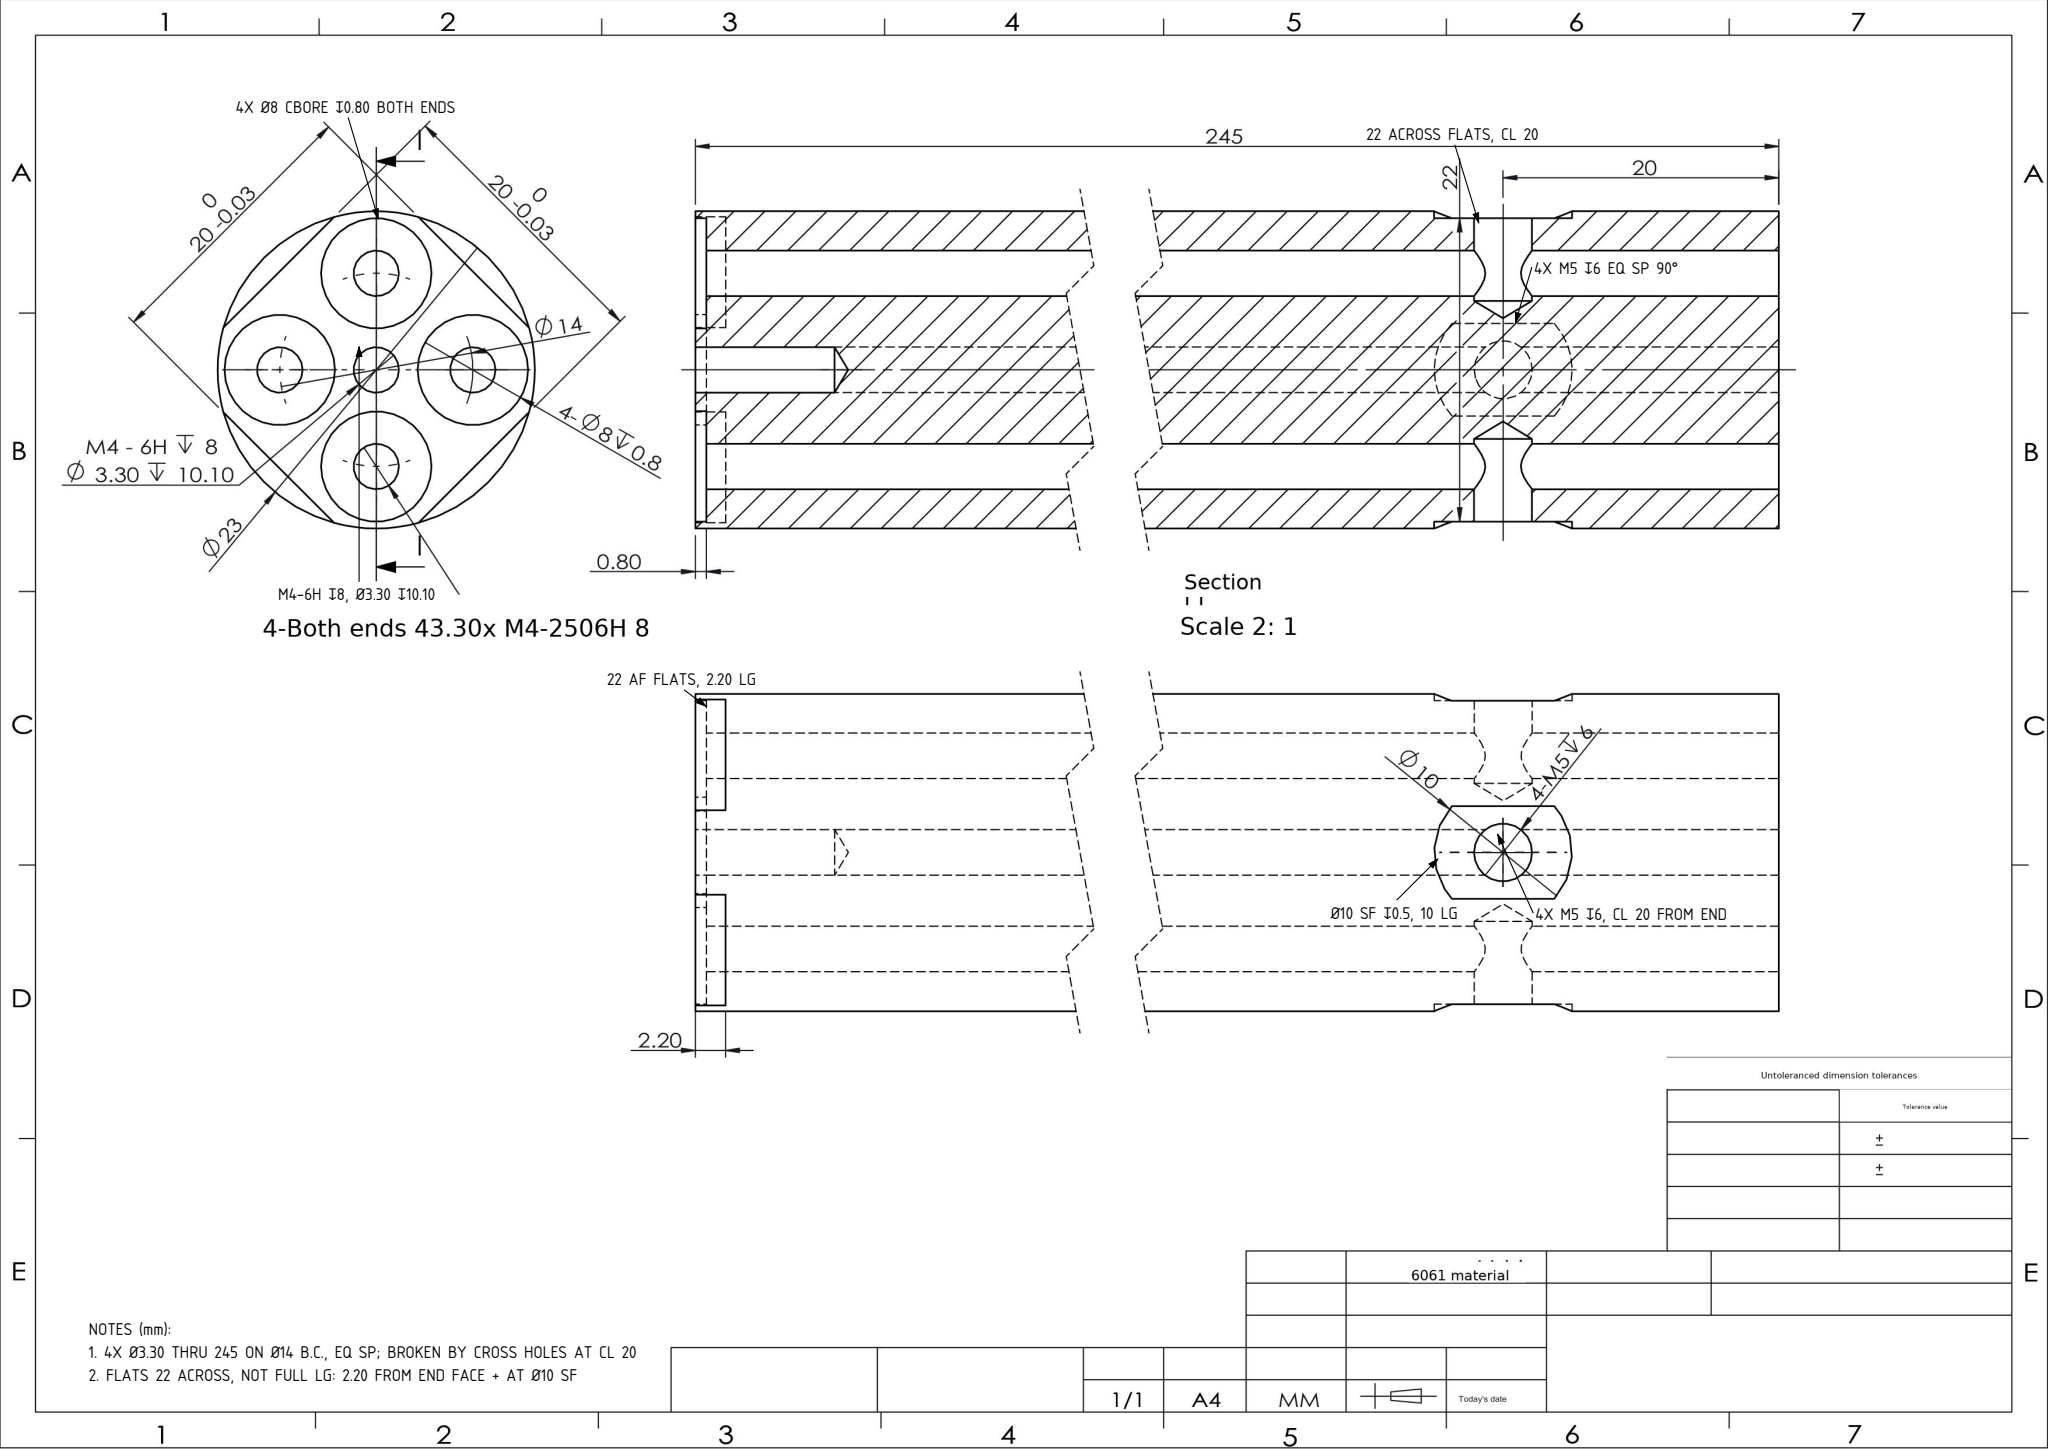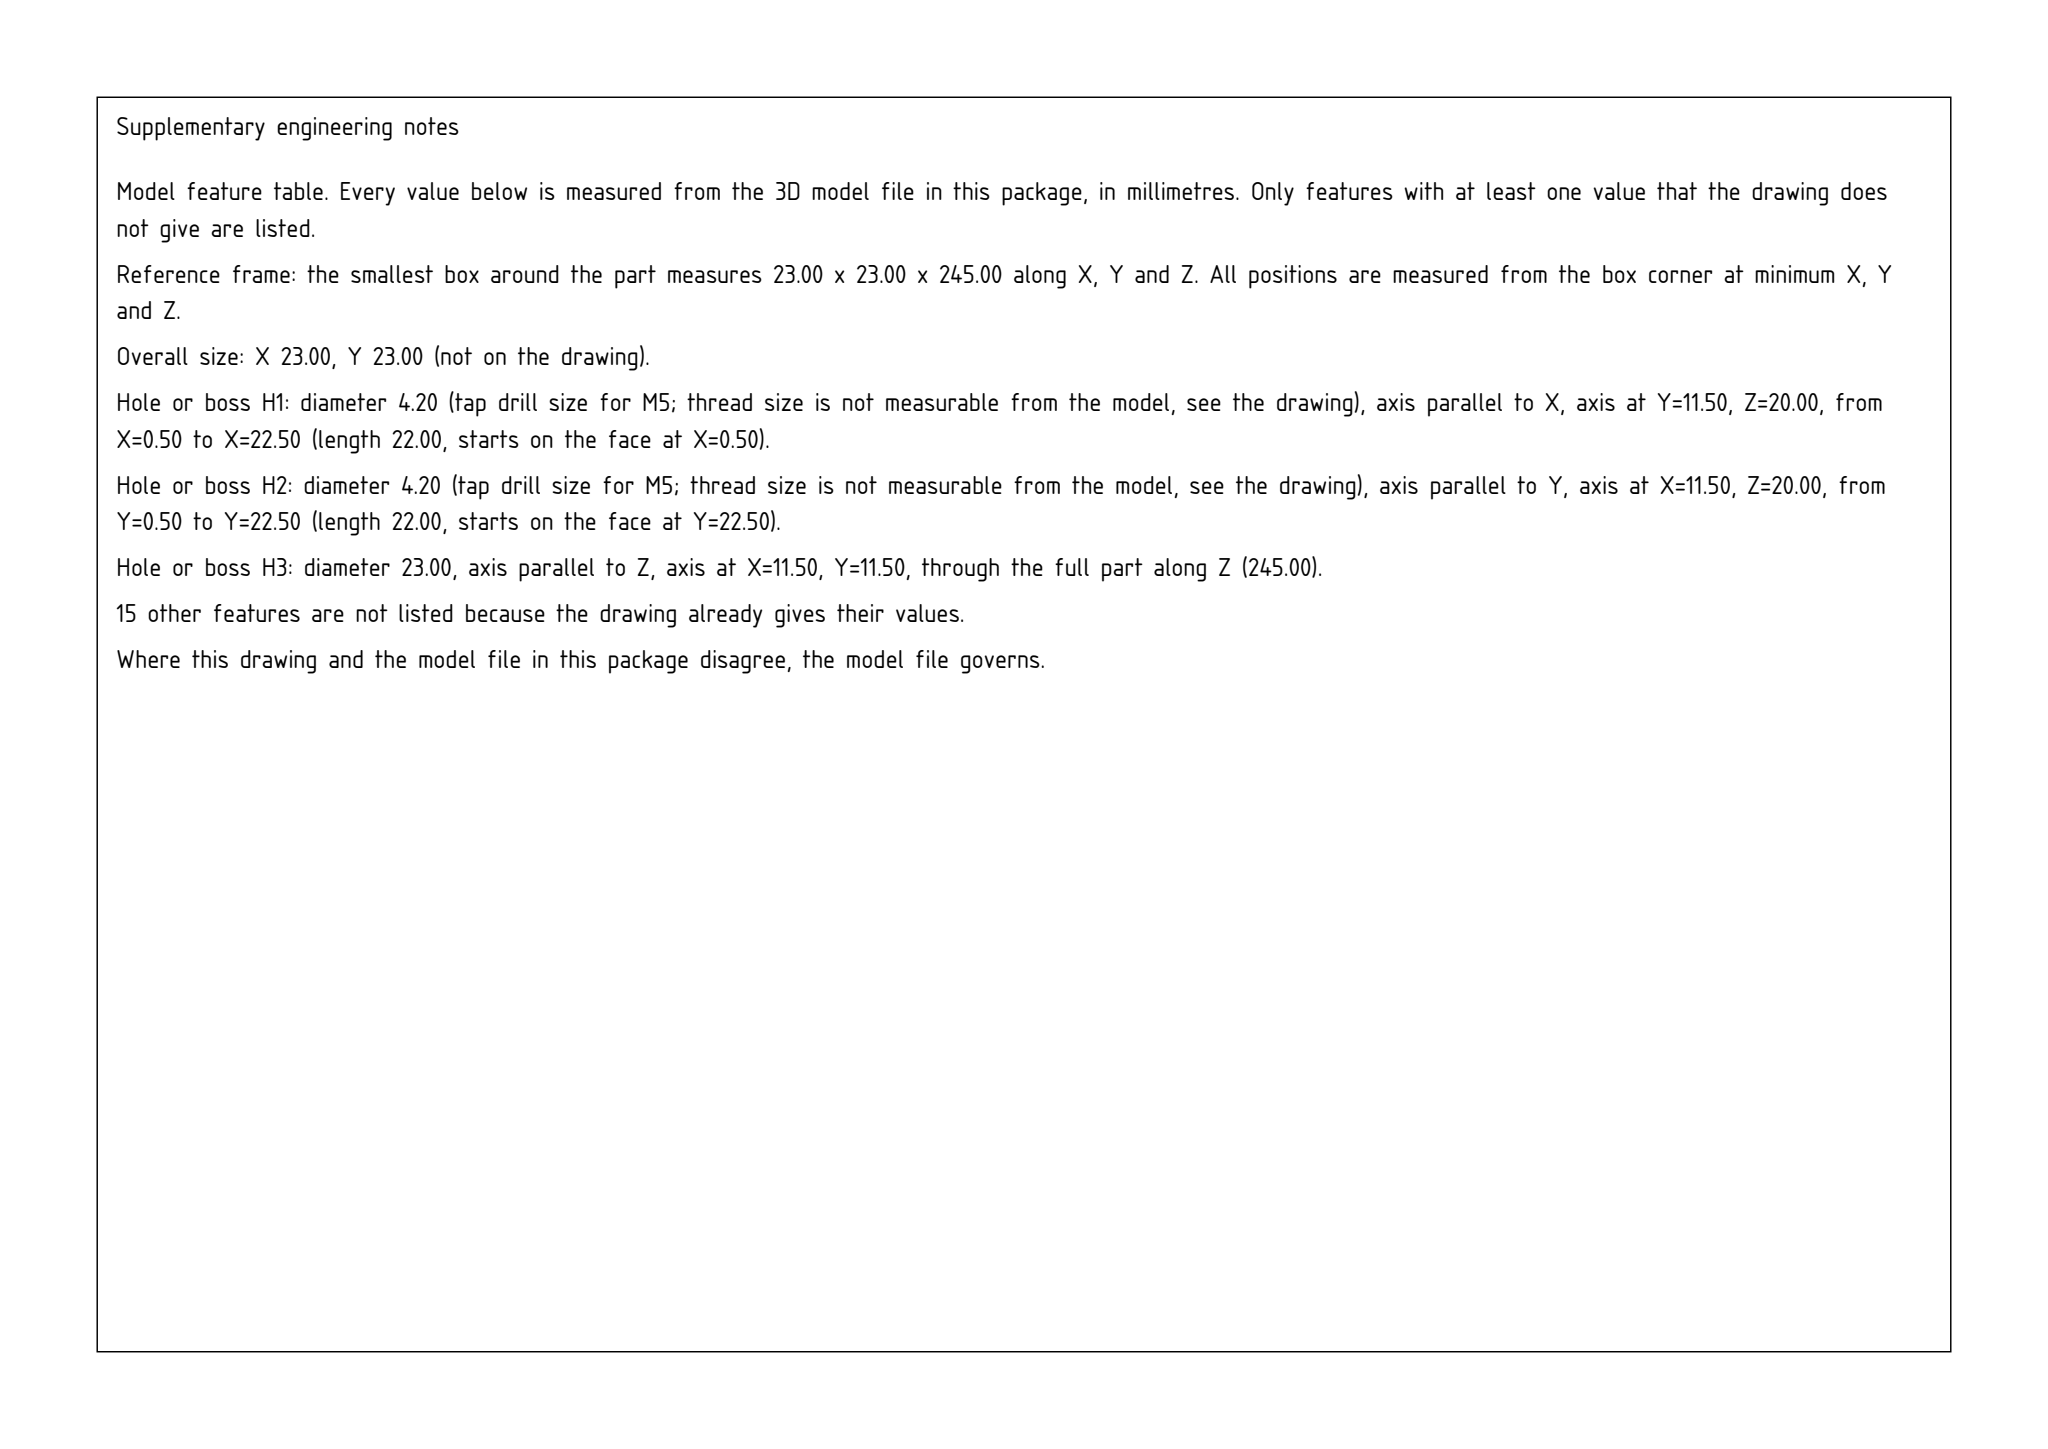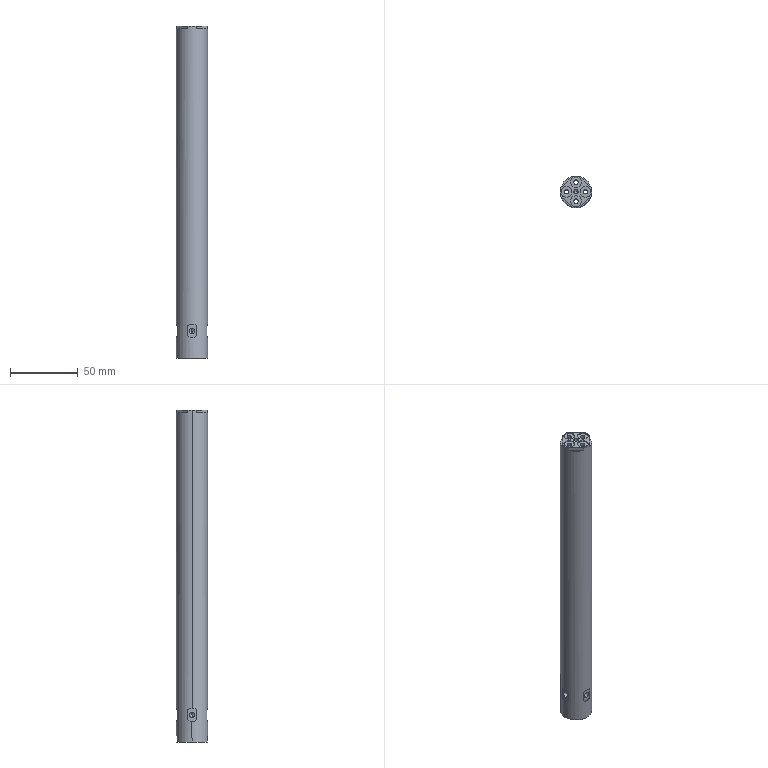Part | SolidWorks | mm | material 6061 | 1 solid | 74 faces | box 23 x 23 x 245 mm | volume 92776 mm3 | cylinder 46 | plane 18 | cone 10 | commonest cylinder face diameters 3.3 x18 10 x10 4.2 x8 8 x8 23 x2
Drawing notes:
4X Ø3.30 THRU 245 ON Ø14 B.C., EQ SP; BROKEN BY CROSS HOLES AT CL 20 | from the solid: Ø3.3 z-cyls at (4.5,11.5),(11.5,4.5),(11.5,18.5),(18.5,11.5): 18.7 lg from z=0 + 222.9 lg from z=245, gap at Ø4.2 cross holes z=17.9-22.1
4X Ø8 CBORE DP0.80 ON Ø14 B.C., EQ SP, BOTH ENDS | from the solid: Ø8.0 z-cyls len 0.8 at the 4 B.C. positions (R7 from axis 11.5,11.5 -> Ø14 B.C.), count 2 ea = z=0 and z=244.2 faces
CTR M4-6H DP8, Ø3.30 DRILL DP10.10, 118° PT, BOTH ENDS | from the solid: Ø3.3 z-cyl at (11.5,11.5) len 10.1, count 2 (one per end); cone 118° ref dia 3.3, count 2
NECK AT CROSS HOLES: 22 ACROSS FLATS, Ø10 SPOTFACE DP0.50 EA FLAT, CL 20 FROM END | from the solid: Planes normal x at 0.5 & 22.5 and normal y at 0.5 & 22.5 (22 across flats); Ø10 x/y cyls len 0.5 at y=11.5 / x=11.5, z=20.0
4X M5 DP6 CROSS HOLES AT CL 20 FROM EA END, Ø4.2 TAP DRILL, 118° PT | from the solid: Ø4.2 x-cyls and y-cyls len 6.0 at z=20.0 through axis 11.5, count 4 ea axis (4 per end); cones 118° ref dia 4.2, count 8
FLAT AT 4X M5: Ø10 SPOTFACE DP 0.5, 10 AXIAL LG, AT 20 STA | from the solid: Ø10 cyls depth 0.5 on x & y at z=20.0; flat planes x/y at 0.5 & 22.5 (0.5 below Ø23)
FLATS 22 ACROSS, NOT FULL LG: 2.20 FROM END FACE + AT Ø10 SF | from the solid: Ø23 OD with planes x=0.5/22.5, y=0.5/22.5 => 22 across flats; z-planes at 242.8 (=245-2.2) x4
4X M5 DP 6 CROSS HOLES EQ SP 90°, IN LINE W/ Ø14 B.C. HOLES | from the solid: Ø4.2 x-axis holes at y=11.5 and y-axis holes at x=11.5, z=20; Ø3.3 B.C. holes at (4.5,11.5),(11.5,4.5),(11.5,18.5),(18.5,11.5)
2.20 = AXIAL LG OF 4X END FLATS, 22 ACROSS FLATS | from the solid: 4 planes at z=242.8 (2.2 from 245 end face) bounding flats at x/y = 0.5 & 22.5
build123d program:
from build123d import *

# Parameters (mm, degrees)
SKETCH1_R             = 11.5
BOSS_EXTRUDE1_DEPTH   = 245
CIRPATTERN1_COUNT     = 4
SKETCH4_R             = 4
CUT_EXTRUDE1_DEPTH    = 0.8
M4_TAPPED_HOLE1_D     = 3.3
M4_TAPPED_HOLE1_DEPTH = 10.1
M4_TAPPED_HOLE1_TIP   = 0.9914
SKETCH7_R             = 18.798
CUT_EXTRUDE2_DEPTH    = 2.2
CUT_EXTRUDE3_START    = 11
SKETCH8_R             = 5
CUT_EXTRUDE3_DEPTH    = 5
CIRPATTERN2_COUNT     = 4


with BuildPart() as part:
    # Sketch1 → Boss-Extrude1 (new body)
    with BuildSketch(Plane.XY):
        Circle(SKETCH1_R)
    extrude(amount=BOSS_EXTRUDE1_DEPTH)

    # Sketch2 → M4 Tapped Hole2 (revolve, cut)
    with BuildSketch(Plane(origin=(0, 7, 0), x_dir=(0, 1, 0), z_dir=(1, 0, 0))):
        Polygon((0, 0), (0, 250.991), (1.65, 250), (1.65, 0), align=None)
    m4_tapped_hole2 = revolve(axis=Axis((0, 7, -6.35), (0, 0, 1)), mode=Mode.SUBTRACT)

    # CirPattern1: M4 Tapped Hole2 ×4 about axis
    cirpattern1_axis = Axis((0, 0, 0), (0, 0, 1))
    for i in range(1, CIRPATTERN1_COUNT):
        add(m4_tapped_hole2.rotate(cirpattern1_axis, i * 360 / CIRPATTERN1_COUNT), mode=Mode.SUBTRACT)

    # Sketch4 → Cut-Extrude1 (cut)
    with BuildSketch(Plane.XY.offset(245)):
        with Locations((7, 0)):
            Circle(SKETCH4_R)
        with Locations((0, -7)):
            Circle(SKETCH4_R)
        with Locations((-7, 0)):
            Circle(SKETCH4_R)
        with Locations((0, 7)):
            Circle(SKETCH4_R)
    extrude(amount=-CUT_EXTRUDE1_DEPTH, mode=Mode.SUBTRACT)

    # M4 Tapped Hole1
    with Locations(Plane.XY.offset(245)):
        with Locations((0, 0)):
            Hole(M4_TAPPED_HOLE1_D / 2, depth=M4_TAPPED_HOLE1_DEPTH)
            with Locations((0, 0, -(M4_TAPPED_HOLE1_DEPTH + M4_TAPPED_HOLE1_TIP / 2))):  # 118° drill point
                Cone(0, M4_TAPPED_HOLE1_D / 2, M4_TAPPED_HOLE1_TIP, mode=Mode.SUBTRACT)

    # Sketch7 → Cut-Extrude2 (cut)
    with BuildSketch(Plane.XY.offset(245)):
        Circle(SKETCH7_R)
        Polygon((0, 14.142), (14.142, 0), (0, -14.142), (-14.142, 0), align=None, mode=Mode.SUBTRACT)
    extrude(amount=-CUT_EXTRUDE2_DEPTH, mode=Mode.SUBTRACT)

    # Sketch8 → Cut-Extrude3 (cut)
    with BuildSketch(Plane(origin=(0, 0, 0), x_dir=(0, 0, -1), z_dir=(1, 0, 0)).offset(CUT_EXTRUDE3_START)):
        with Locations((-20, 0)):
            Circle(SKETCH8_R)
    cut_extrude3 = extrude(amount=CUT_EXTRUDE3_DEPTH, mode=Mode.SUBTRACT)

    # Sketch9 → M5 Tapped Hole2 (revolve, cut)
    with BuildSketch(Plane(origin=(11, 0, 20), x_dir=(0, 0, -1), z_dir=(0, 1, 0))):
        Polygon((0, 0), (0, 7.262), (2.1, 6), (2.1, 0), align=None)
    m5_tapped_hole2 = revolve(axis=Axis((17.35, 0, 20), (-1, 0, 0)), mode=Mode.SUBTRACT)

    # CirPattern2: Cut-Extrude3, M5 Tapped Hole2 ×4 about axis
    cirpattern2_axis = Axis((0, 0, 0), (0, 0, 1))
    add([cut_extrude3.rotate(cirpattern2_axis, i * 360 / CIRPATTERN2_COUNT) for i in range(1, CIRPATTERN2_COUNT)], mode=Mode.SUBTRACT)
    add([m5_tapped_hole2.rotate(cirpattern2_axis, i * 360 / CIRPATTERN2_COUNT) for i in range(1, CIRPATTERN2_COUNT)], mode=Mode.SUBTRACT)


solid = part.part